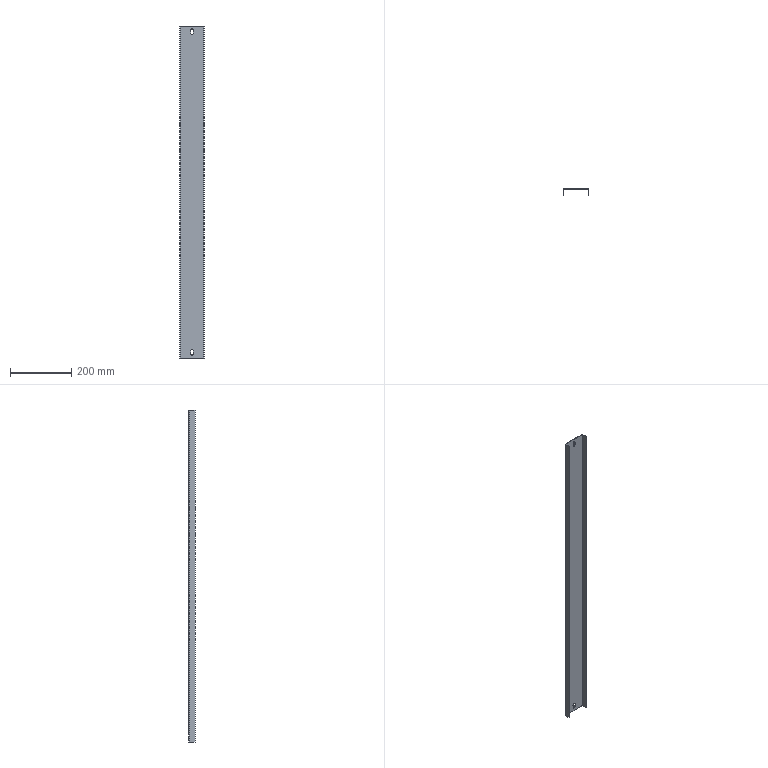Component | SolidWorks | MountingPlate-1 | 1 solid | 32 faces | box 81.5 x 20 x 1085 mm | volume 191237 mm3 | plane 22 | cylinder 10 | commonest cylinder face diameters 9 x6 3.2 x2 0.2 x2
STEP:
#1=COLOUR_RGB('',0.7922,0.8196,0.9333);
#2=FILL_AREA_STYLE_COLOUR('',#1);
#3=FILL_AREA_STYLE('',(#2));
#4=SURFACE_STYLE_FILL_AREA(#3);
#5=SURFACE_SIDE_STYLE('',(#4));
#6=SURFACE_STYLE_USAGE(.BOTH.,#5);
#7=PRESENTATION_STYLE_ASSIGNMENT((#6));
#8=CARTESIAN_POINT('',(11.302,-36.434,95.784));
#9=VERTEX_POINT('',#8);
#10=CARTESIAN_POINT('',(11.125,-36.434,95.607));
#11=VERTEX_POINT('',#10);
#12=CARTESIAN_POINT('',(11.302,-36.434,95.607));
#13=DIRECTION('',(0.,-1.,-0.));
#14=DIRECTION('',(0.,0.,1.));
#15=AXIS2_PLACEMENT_3D('',#12,#13,#14);
#16=CIRCLE('',#15,0.1772);
#17=EDGE_CURVE('',#9,#11,#16,.T.);
#18=ORIENTED_EDGE('',*,*,#17,.F.);
#19=CARTESIAN_POINT('',(11.302,-36.493,95.784));
#20=VERTEX_POINT('',#19);
#21=CARTESIAN_POINT('',(11.302,-36.434,95.784));
#22=DIRECTION('',(0.,-1.,-0.));
#23=VECTOR('',#22,39.37);
#24=LINE('',#21,#23);
#25=EDGE_CURVE('',#9,#20,#24,.T.);
#26=ORIENTED_EDGE('',*,*,#25,.T.);
#27=CARTESIAN_POINT('',(11.125,-36.493,95.607));
#28=VERTEX_POINT('',#27);
#29=CARTESIAN_POINT('',(11.302,-36.493,95.607));
#30=DIRECTION('',(0.,-1.,-0.));
#31=DIRECTION('',(0.,0.,1.));
#32=AXIS2_PLACEMENT_3D('',#29,#30,#31);
#33=CIRCLE('',#32,0.1772);
#34=EDGE_CURVE('',#20,#28,#33,.T.);
#35=ORIENTED_EDGE('',*,*,#34,.T.);
#36=CARTESIAN_POINT('',(11.125,-36.434,95.607));
#37=DIRECTION('',(0.,-1.,-0.));
#38=VECTOR('',#37,39.37);
#39=LINE('',#36,#38);
#40=EDGE_CURVE('',#11,#28,#39,.T.);
#41=ORIENTED_EDGE('',*,*,#40,.F.);
#42=EDGE_LOOP('',(#18,#26,#35,#41));
#43=FACE_OUTER_BOUND('',#42,.T.);
#44=CARTESIAN_POINT('',(11.302,-36.434,95.607));
#45=DIRECTION('',(0.,-1.,-0.));
#46=DIRECTION('',(0.,0.,1.));
#47=AXIS2_PLACEMENT_3D('',#44,#45,#46);
#48=CYLINDRICAL_SURFACE('',#47,0.1772);
#49=ADVANCED_FACE('',(#43),#48,.F.);
#50=CARTESIAN_POINT('',(11.302,-36.434,54.532));
#51=VERTEX_POINT('',#50);
#52=CARTESIAN_POINT('',(11.125,-36.434,54.355));
#53=VERTEX_POINT('',#52);
#54=CARTESIAN_POINT('',(11.302,-36.434,54.355));
#55=DIRECTION('',(0.,-1.,-0.));
#56=DIRECTION('',(0.,0.,1.));
#57=AXIS2_PLACEMENT_3D('',#54,#55,#56);
#58=CIRCLE('',#57,0.1772);
#59=EDGE_CURVE('',#51,#53,#58,.T.);
#60=ORIENTED_EDGE('',*,*,#59,.F.);
#61=CARTESIAN_POINT('',(11.302,-36.493,54.532));
#62=VERTEX_POINT('',#61);
#63=CARTESIAN_POINT('',(11.302,-36.434,54.532));
#64=DIRECTION('',(0.,-1.,-0.));
#65=VECTOR('',#64,39.37);
#66=LINE('',#63,#65);
#67=EDGE_CURVE('',#51,#62,#66,.T.);
#68=ORIENTED_EDGE('',*,*,#67,.T.);
#69=CARTESIAN_POINT('',(11.125,-36.493,54.355));
#70=VERTEX_POINT('',#69);
#71=CARTESIAN_POINT('',(11.302,-36.493,54.355));
#72=DIRECTION('',(0.,-1.,-0.));
#73=DIRECTION('',(0.,0.,1.));
#74=AXIS2_PLACEMENT_3D('',#71,#72,#73);
#75=CIRCLE('',#74,0.1772);
#76=EDGE_CURVE('',#62,#70,#75,.T.);
#77=ORIENTED_EDGE('',*,*,#76,.T.);
#78=CARTESIAN_POINT('',(11.125,-36.434,54.355));
#79=DIRECTION('',(0.,-1.,-0.));
#80=VECTOR('',#79,39.37);
#81=LINE('',#78,#80);
#82=EDGE_CURVE('',#53,#70,#81,.T.);
#83=ORIENTED_EDGE('',*,*,#82,.F.);
#84=EDGE_LOOP('',(#60,#68,#77,#83));
#85=FACE_OUTER_BOUND('',#84,.T.);
#86=CARTESIAN_POINT('',(11.302,-36.434,54.355));
#87=DIRECTION('',(0.,-1.,-0.));
#88=DIRECTION('',(0.,0.,1.));
#89=AXIS2_PLACEMENT_3D('',#86,#87,#88);
#90=CYLINDRICAL_SURFACE('',#89,0.1772);
#91=ADVANCED_FACE('',(#85),#90,.F.);
#92=CARTESIAN_POINT('',(11.48,-36.493,54.));
#93=VERTEX_POINT('',#92);
#94=CARTESIAN_POINT('',(11.48,-36.493,54.355));
#95=VERTEX_POINT('',#94);
#96=CARTESIAN_POINT('',(11.48,-36.493,54.355));
#97=DIRECTION('',(0.,-0.,1.));
#98=VECTOR('',#97,39.37);
#99=LINE('',#96,#98);
#100=EDGE_CURVE('',#93,#95,#99,.T.);
#101=ORIENTED_EDGE('',*,*,#100,.F.);
#102=CARTESIAN_POINT('',(11.125,-36.493,54.));
#103=VERTEX_POINT('',#102);
#104=CARTESIAN_POINT('',(11.302,-36.493,54.));
#105=DIRECTION('',(0.,-1.,-0.));
#106=DIRECTION('',(0.,0.,1.));
#107=AXIS2_PLACEMENT_3D('',#104,#105,#106);
#108=CIRCLE('',#107,0.1772);
#109=EDGE_CURVE('',#103,#93,#108,.T.);
#110=ORIENTED_EDGE('',*,*,#109,.F.);
#111=CARTESIAN_POINT('',(11.125,-36.493,54.355));
#112=DIRECTION('',(-0.,0.,-1.));
#113=VECTOR('',#112,39.37);
#114=LINE('',#111,#113);
#115=EDGE_CURVE('',#70,#103,#114,.T.);
#116=ORIENTED_EDGE('',*,*,#115,.F.);
#117=ORIENTED_EDGE('',*,*,#76,.F.);
#118=CARTESIAN_POINT('',(11.302,-36.493,54.355));
#119=DIRECTION('',(0.,-1.,-0.));
#120=DIRECTION('',(0.,0.,1.));
#121=AXIS2_PLACEMENT_3D('',#118,#119,#120);
#122=CIRCLE('',#121,0.1772);
#123=EDGE_CURVE('',#95,#62,#122,.T.);
#124=ORIENTED_EDGE('',*,*,#123,.F.);
#125=EDGE_LOOP('',(#101,#110,#116,#117,#124));
#126=FACE_BOUND('',#125,.T.);
#127=CARTESIAN_POINT('',(11.48,-36.493,95.252));
#128=VERTEX_POINT('',#127);
#129=CARTESIAN_POINT('',(11.48,-36.493,95.607));
#130=VERTEX_POINT('',#129);
#131=CARTESIAN_POINT('',(11.48,-36.493,95.607));
#132=DIRECTION('',(-0.,-0.,1.));
#133=VECTOR('',#132,39.37);
#134=LINE('',#131,#133);
#135=EDGE_CURVE('',#128,#130,#134,.T.);
#136=ORIENTED_EDGE('',*,*,#135,.F.);
#137=CARTESIAN_POINT('',(11.125,-36.493,95.252));
#138=VERTEX_POINT('',#137);
#139=CARTESIAN_POINT('',(11.302,-36.493,95.252));
#140=DIRECTION('',(0.,-1.,-0.));
#141=DIRECTION('',(0.,0.,1.));
#142=AXIS2_PLACEMENT_3D('',#139,#140,#141);
#143=CIRCLE('',#142,0.1772);
#144=EDGE_CURVE('',#138,#128,#143,.T.);
#145=ORIENTED_EDGE('',*,*,#144,.F.);
#146=CARTESIAN_POINT('',(11.125,-36.493,95.607));
#147=DIRECTION('',(-0.,0.,-1.));
#148=VECTOR('',#147,39.37);
#149=LINE('',#146,#148);
#150=EDGE_CURVE('',#28,#138,#149,.T.);
#151=ORIENTED_EDGE('',*,*,#150,.F.);
#152=ORIENTED_EDGE('',*,*,#34,.F.);
#153=CARTESIAN_POINT('',(11.302,-36.493,95.607));
#154=DIRECTION('',(0.,-1.,-0.));
#155=DIRECTION('',(0.,0.,1.));
#156=AXIS2_PLACEMENT_3D('',#153,#154,#155);
#157=CIRCLE('',#156,0.1772);
#158=EDGE_CURVE('',#130,#20,#157,.T.);
#159=ORIENTED_EDGE('',*,*,#158,.F.);
#160=EDGE_LOOP('',(#136,#145,#151,#152,#159));
#161=FACE_BOUND('',#160,.T.);
#162=CARTESIAN_POINT('',(9.761,-36.493,53.445));
#163=VERTEX_POINT('',#162);
#164=CARTESIAN_POINT('',(12.844,-36.493,53.445));
#165=VERTEX_POINT('',#164);
#166=CARTESIAN_POINT('',(13.604,-36.493,53.445));
#167=DIRECTION('',(1.,0.,-0.));
#168=VECTOR('',#167,39.37);
#169=LINE('',#166,#168);
#170=EDGE_CURVE('',#163,#165,#169,.T.);
#171=ORIENTED_EDGE('',*,*,#170,.T.);
#172=CARTESIAN_POINT('',(12.844,-36.493,96.162));
#173=VERTEX_POINT('',#172);
#174=CARTESIAN_POINT('',(12.844,-36.493,-1322.049));
#175=DIRECTION('',(0.,-0.,1.));
#176=VECTOR('',#175,39.37);
#177=LINE('',#174,#176);
#178=EDGE_CURVE('',#165,#173,#177,.T.);
#179=ORIENTED_EDGE('',*,*,#178,.T.);
#180=CARTESIAN_POINT('',(9.761,-36.493,96.162));
#181=VERTEX_POINT('',#180);
#182=CARTESIAN_POINT('',(9.001,-36.493,96.162));
#183=DIRECTION('',(-1.,-0.,0.));
#184=VECTOR('',#183,39.37);
#185=LINE('',#182,#184);
#186=EDGE_CURVE('',#173,#181,#185,.T.);
#187=ORIENTED_EDGE('',*,*,#186,.T.);
#188=CARTESIAN_POINT('',(9.761,-36.493,-1322.049));
#189=DIRECTION('',(0.,-0.,1.));
#190=VECTOR('',#189,39.37);
#191=LINE('',#188,#190);
#192=EDGE_CURVE('',#163,#181,#191,.T.);
#193=ORIENTED_EDGE('',*,*,#192,.F.);
#194=EDGE_LOOP('',(#171,#179,#187,#193));
#195=FACE_OUTER_BOUND('',#194,.T.);
#196=CARTESIAN_POINT('',(320.089,-36.493,-1322.049));
#197=DIRECTION('',(-0.,1.,0.));
#198=DIRECTION('',(-0.,0.,-1.));
#199=AXIS2_PLACEMENT_3D('',#196,#197,#198);
#200=PLANE('',#199);
#201=ADVANCED_FACE('',(#126,#161,#195),#200,.F.);
#202=CARTESIAN_POINT('',(12.844,-36.434,53.445));
#203=VERTEX_POINT('',#202);
#204=CARTESIAN_POINT('',(12.844,-36.434,53.445));
#205=DIRECTION('',(-0.,1.,0.));
#206=VECTOR('',#205,39.37);
#207=LINE('',#204,#206);
#208=EDGE_CURVE('',#165,#203,#207,.T.);
#209=ORIENTED_EDGE('',*,*,#208,.F.);
#210=ORIENTED_EDGE('',*,*,#170,.F.);
#211=CARTESIAN_POINT('',(9.761,-36.434,53.445));
#212=VERTEX_POINT('',#211);
#213=CARTESIAN_POINT('',(9.761,-36.434,53.445));
#214=DIRECTION('',(-0.,1.,0.));
#215=VECTOR('',#214,39.37);
#216=LINE('',#213,#215);
#217=EDGE_CURVE('',#163,#212,#216,.T.);
#218=ORIENTED_EDGE('',*,*,#217,.T.);
#219=CARTESIAN_POINT('',(13.604,-36.434,53.445));
#220=DIRECTION('',(1.,0.,-0.));
#221=VECTOR('',#220,39.37);
#222=LINE('',#219,#221);
#223=EDGE_CURVE('',#212,#203,#222,.T.);
#224=ORIENTED_EDGE('',*,*,#223,.T.);
#225=EDGE_LOOP('',(#209,#210,#218,#224));
#226=FACE_OUTER_BOUND('',#225,.T.);
#227=CARTESIAN_POINT('',(13.604,-36.434,53.445));
#228=DIRECTION('',(-0.,0.,-1.));
#229=DIRECTION('',(0.,-1.,-0.));
#230=AXIS2_PLACEMENT_3D('',#227,#228,#229);
#231=PLANE('',#230);
#232=ADVANCED_FACE('',(#226),#231,.T.);
#233=CARTESIAN_POINT('',(12.844,-36.434,96.162));
#234=VERTEX_POINT('',#233);
#235=CARTESIAN_POINT('',(12.844,-36.434,96.162));
#236=DIRECTION('',(0.,-1.,-0.));
#237=VECTOR('',#236,39.37);
#238=LINE('',#235,#237);
#239=EDGE_CURVE('',#234,#173,#238,.T.);
#240=ORIENTED_EDGE('',*,*,#239,.F.);
#241=CARTESIAN_POINT('',(9.761,-36.434,96.162));
#242=VERTEX_POINT('',#241);
#243=CARTESIAN_POINT('',(9.001,-36.434,96.162));
#244=DIRECTION('',(-1.,-0.,0.));
#245=VECTOR('',#244,39.37);
#246=LINE('',#243,#245);
#247=EDGE_CURVE('',#234,#242,#246,.T.);
#248=ORIENTED_EDGE('',*,*,#247,.T.);
#249=CARTESIAN_POINT('',(9.761,-36.434,96.162));
#250=DIRECTION('',(0.,-1.,-0.));
#251=VECTOR('',#250,39.37);
#252=LINE('',#249,#251);
#253=EDGE_CURVE('',#242,#181,#252,.T.);
#254=ORIENTED_EDGE('',*,*,#253,.T.);
#255=ORIENTED_EDGE('',*,*,#186,.F.);
#256=EDGE_LOOP('',(#240,#248,#254,#255));
#257=FACE_OUTER_BOUND('',#256,.T.);
#258=CARTESIAN_POINT('',(9.001,-36.434,96.162));
#259=DIRECTION('',(0.,-0.,1.));
#260=DIRECTION('',(-0.,1.,0.));
#261=AXIS2_PLACEMENT_3D('',#258,#259,#260);
#262=PLANE('',#261);
#263=ADVANCED_FACE('',(#257),#262,.T.);
#264=CARTESIAN_POINT('',(12.844,-36.434,-1322.049));
#265=DIRECTION('',(0.,-0.,1.));
#266=VECTOR('',#265,39.37);
#267=LINE('',#264,#266);
#268=EDGE_CURVE('',#203,#234,#267,.T.);
#269=ORIENTED_EDGE('',*,*,#268,.F.);
#270=ORIENTED_EDGE('',*,*,#223,.F.);
#271=CARTESIAN_POINT('',(9.761,-36.434,-1322.049));
#272=DIRECTION('',(0.,-0.,1.));
#273=VECTOR('',#272,39.37);
#274=LINE('',#271,#273);
#275=EDGE_CURVE('',#212,#242,#274,.T.);
#276=ORIENTED_EDGE('',*,*,#275,.T.);
#277=ORIENTED_EDGE('',*,*,#247,.F.);
#278=EDGE_LOOP('',(#269,#270,#276,#277));
#279=FACE_OUTER_BOUND('',#278,.T.);
#280=CARTESIAN_POINT('',(11.125,-36.434,95.252));
#281=VERTEX_POINT('',#280);
#282=CARTESIAN_POINT('',(11.48,-36.434,95.252));
#283=VERTEX_POINT('',#282);
#284=CARTESIAN_POINT('',(11.302,-36.434,95.252));
#285=DIRECTION('',(0.,-1.,-0.));
#286=DIRECTION('',(0.,0.,1.));
#287=AXIS2_PLACEMENT_3D('',#284,#285,#286);
#288=CIRCLE('',#287,0.1772);
#289=EDGE_CURVE('',#281,#283,#288,.T.);
#290=ORIENTED_EDGE('',*,*,#289,.T.);
#291=CARTESIAN_POINT('',(11.48,-36.434,95.607));
#292=VERTEX_POINT('',#291);
#293=CARTESIAN_POINT('',(11.48,-36.434,95.607));
#294=DIRECTION('',(-0.,-0.,1.));
#295=VECTOR('',#294,39.37);
#296=LINE('',#293,#295);
#297=EDGE_CURVE('',#283,#292,#296,.T.);
#298=ORIENTED_EDGE('',*,*,#297,.T.);
#299=CARTESIAN_POINT('',(11.302,-36.434,95.607));
#300=DIRECTION('',(0.,-1.,-0.));
#301=DIRECTION('',(0.,0.,1.));
#302=AXIS2_PLACEMENT_3D('',#299,#300,#301);
#303=CIRCLE('',#302,0.1772);
#304=EDGE_CURVE('',#292,#9,#303,.T.);
#305=ORIENTED_EDGE('',*,*,#304,.T.);
#306=ORIENTED_EDGE('',*,*,#17,.T.);
#307=CARTESIAN_POINT('',(11.125,-36.434,95.607));
#308=DIRECTION('',(-0.,0.,-1.));
#309=VECTOR('',#308,39.37);
#310=LINE('',#307,#309);
#311=EDGE_CURVE('',#11,#281,#310,.T.);
#312=ORIENTED_EDGE('',*,*,#311,.T.);
#313=EDGE_LOOP('',(#290,#298,#305,#306,#312));
#314=FACE_BOUND('',#313,.T.);
#315=CARTESIAN_POINT('',(11.125,-36.434,54.));
#316=VERTEX_POINT('',#315);
#317=CARTESIAN_POINT('',(11.48,-36.434,54.));
#318=VERTEX_POINT('',#317);
#319=CARTESIAN_POINT('',(11.302,-36.434,54.));
#320=DIRECTION('',(0.,-1.,-0.));
#321=DIRECTION('',(0.,0.,1.));
#322=AXIS2_PLACEMENT_3D('',#319,#320,#321);
#323=CIRCLE('',#322,0.1772);
#324=EDGE_CURVE('',#316,#318,#323,.T.);
#325=ORIENTED_EDGE('',*,*,#324,.T.);
#326=CARTESIAN_POINT('',(11.48,-36.434,54.355));
#327=VERTEX_POINT('',#326);
#328=CARTESIAN_POINT('',(11.48,-36.434,54.355));
#329=DIRECTION('',(0.,-0.,1.));
#330=VECTOR('',#329,39.37);
#331=LINE('',#328,#330);
#332=EDGE_CURVE('',#318,#327,#331,.T.);
#333=ORIENTED_EDGE('',*,*,#332,.T.);
#334=CARTESIAN_POINT('',(11.302,-36.434,54.355));
#335=DIRECTION('',(0.,-1.,-0.));
#336=DIRECTION('',(0.,0.,1.));
#337=AXIS2_PLACEMENT_3D('',#334,#335,#336);
#338=CIRCLE('',#337,0.1772);
#339=EDGE_CURVE('',#327,#51,#338,.T.);
#340=ORIENTED_EDGE('',*,*,#339,.T.);
#341=ORIENTED_EDGE('',*,*,#59,.T.);
#342=CARTESIAN_POINT('',(11.125,-36.434,54.355));
#343=DIRECTION('',(-0.,0.,-1.));
#344=VECTOR('',#343,39.37);
#345=LINE('',#342,#344);
#346=EDGE_CURVE('',#53,#316,#345,.T.);
#347=ORIENTED_EDGE('',*,*,#346,.T.);
#348=EDGE_LOOP('',(#325,#333,#340,#341,#347));
#349=FACE_BOUND('',#348,.T.);
#350=CARTESIAN_POINT('',(320.089,-36.434,-1322.049));
#351=DIRECTION('',(-0.,1.,0.));
#352=DIRECTION('',(-0.,0.,-1.));
#353=AXIS2_PLACEMENT_3D('',#350,#351,#352);
#354=PLANE('',#353);
#355=ADVANCED_FACE('',(#279,#314,#349),#354,.T.);
#356=ORIENTED_EDGE('',*,*,#109,.T.);
#357=CARTESIAN_POINT('',(11.48,-36.434,54.));
#358=DIRECTION('',(0.,-1.,-0.));
#359=VECTOR('',#358,39.37);
#360=LINE('',#357,#359);
#361=EDGE_CURVE('',#318,#93,#360,.T.);
#362=ORIENTED_EDGE('',*,*,#361,.F.);
#363=ORIENTED_EDGE('',*,*,#324,.F.);
#364=CARTESIAN_POINT('',(11.125,-36.434,54.));
#365=DIRECTION('',(0.,-1.,-0.));
#366=VECTOR('',#365,39.37);
#367=LINE('',#364,#366);
#368=EDGE_CURVE('',#316,#103,#367,.T.);
#369=ORIENTED_EDGE('',*,*,#368,.T.);
#370=EDGE_LOOP('',(#356,#362,#363,#369));
#371=FACE_OUTER_BOUND('',#370,.T.);
#372=CARTESIAN_POINT('',(11.302,-36.434,54.));
#373=DIRECTION('',(0.,-1.,-0.));
#374=DIRECTION('',(0.,0.,1.));
#375=AXIS2_PLACEMENT_3D('',#372,#373,#374);
#376=CYLINDRICAL_SURFACE('',#375,0.1772);
#377=ADVANCED_FACE('',(#371),#376,.F.);
#378=ORIENTED_EDGE('',*,*,#115,.T.);
#379=ORIENTED_EDGE('',*,*,#368,.F.);
#380=ORIENTED_EDGE('',*,*,#346,.F.);
#381=ORIENTED_EDGE('',*,*,#82,.T.);
#382=EDGE_LOOP('',(#378,#379,#380,#381));
#383=FACE_OUTER_BOUND('',#382,.T.);
#384=CARTESIAN_POINT('',(11.125,-36.434,54.355));
#385=DIRECTION('',(-1.,-0.,0.));
#386=DIRECTION('',(0.,-1.,-0.));
#387=AXIS2_PLACEMENT_3D('',#384,#385,#386);
#388=PLANE('',#387);
#389=ADVANCED_FACE('',(#383),#388,.F.);
#390=ORIENTED_EDGE('',*,*,#67,.F.);
#391=ORIENTED_EDGE('',*,*,#339,.F.);
#392=CARTESIAN_POINT('',(11.48,-36.434,54.355));
#393=DIRECTION('',(0.,-1.,-0.));
#394=VECTOR('',#393,39.37);
#395=LINE('',#392,#394);
#396=EDGE_CURVE('',#327,#95,#395,.T.);
#397=ORIENTED_EDGE('',*,*,#396,.T.);
#398=ORIENTED_EDGE('',*,*,#123,.T.);
#399=EDGE_LOOP('',(#390,#391,#397,#398));
#400=FACE_OUTER_BOUND('',#399,.T.);
#401=CARTESIAN_POINT('',(11.302,-36.434,54.355));
#402=DIRECTION('',(0.,-1.,-0.));
#403=DIRECTION('',(0.,0.,1.));
#404=AXIS2_PLACEMENT_3D('',#401,#402,#403);
#405=CYLINDRICAL_SURFACE('',#404,0.1772);
#406=ADVANCED_FACE('',(#400),#405,.F.);
#407=ORIENTED_EDGE('',*,*,#100,.T.);
#408=ORIENTED_EDGE('',*,*,#396,.F.);
#409=ORIENTED_EDGE('',*,*,#332,.F.);
#410=ORIENTED_EDGE('',*,*,#361,.T.);
#411=EDGE_LOOP('',(#407,#408,#409,#410));
#412=FACE_OUTER_BOUND('',#411,.T.);
#413=CARTESIAN_POINT('',(11.48,-36.434,54.355));
#414=DIRECTION('',(1.,0.,-0.));
#415=DIRECTION('',(-0.,1.,0.));
#416=AXIS2_PLACEMENT_3D('',#413,#414,#415);
#417=PLANE('',#416);
#418=ADVANCED_FACE('',(#412),#417,.F.);
#419=ORIENTED_EDGE('',*,*,#144,.T.);
#420=CARTESIAN_POINT('',(11.48,-36.434,95.252));
#421=DIRECTION('',(0.,-1.,-0.));
#422=VECTOR('',#421,39.37);
#423=LINE('',#420,#422);
#424=EDGE_CURVE('',#283,#128,#423,.T.);
#425=ORIENTED_EDGE('',*,*,#424,.F.);
#426=ORIENTED_EDGE('',*,*,#289,.F.);
#427=CARTESIAN_POINT('',(11.125,-36.434,95.252));
#428=DIRECTION('',(0.,-1.,-0.));
#429=VECTOR('',#428,39.37);
#430=LINE('',#427,#429);
#431=EDGE_CURVE('',#281,#138,#430,.T.);
#432=ORIENTED_EDGE('',*,*,#431,.T.);
#433=EDGE_LOOP('',(#419,#425,#426,#432));
#434=FACE_OUTER_BOUND('',#433,.T.);
#435=CARTESIAN_POINT('',(11.302,-36.434,95.252));
#436=DIRECTION('',(0.,-1.,-0.));
#437=DIRECTION('',(0.,0.,1.));
#438=AXIS2_PLACEMENT_3D('',#435,#436,#437);
#439=CYLINDRICAL_SURFACE('',#438,0.1772);
#440=ADVANCED_FACE('',(#434),#439,.F.);
#441=ORIENTED_EDGE('',*,*,#150,.T.);
#442=ORIENTED_EDGE('',*,*,#431,.F.);
#443=ORIENTED_EDGE('',*,*,#311,.F.);
#444=ORIENTED_EDGE('',*,*,#40,.T.);
#445=EDGE_LOOP('',(#441,#442,#443,#444));
#446=FACE_OUTER_BOUND('',#445,.T.);
#447=CARTESIAN_POINT('',(11.125,-36.434,95.607));
#448=DIRECTION('',(-1.,-0.,0.));
#449=DIRECTION('',(0.,-1.,-0.));
#450=AXIS2_PLACEMENT_3D('',#447,#448,#449);
#451=PLANE('',#450);
#452=ADVANCED_FACE('',(#446),#451,.F.);
#453=ORIENTED_EDGE('',*,*,#25,.F.);
#454=ORIENTED_EDGE('',*,*,#304,.F.);
#455=CARTESIAN_POINT('',(11.48,-36.434,95.607));
#456=DIRECTION('',(0.,-1.,-0.));
#457=VECTOR('',#456,39.37);
#458=LINE('',#455,#457);
#459=EDGE_CURVE('',#292,#130,#458,.T.);
#460=ORIENTED_EDGE('',*,*,#459,.T.);
#461=ORIENTED_EDGE('',*,*,#158,.T.);
#462=EDGE_LOOP('',(#453,#454,#460,#461));
#463=FACE_OUTER_BOUND('',#462,.T.);
#464=CARTESIAN_POINT('',(11.302,-36.434,95.607));
#465=DIRECTION('',(0.,-1.,-0.));
#466=DIRECTION('',(0.,0.,1.));
#467=AXIS2_PLACEMENT_3D('',#464,#465,#466);
#468=CYLINDRICAL_SURFACE('',#467,0.1772);
#469=ADVANCED_FACE('',(#463),#468,.F.);
#470=ORIENTED_EDGE('',*,*,#135,.T.);
#471=ORIENTED_EDGE('',*,*,#459,.F.);
#472=ORIENTED_EDGE('',*,*,#297,.F.);
#473=ORIENTED_EDGE('',*,*,#424,.T.);
#474=EDGE_LOOP('',(#470,#471,#472,#473));
#475=FACE_OUTER_BOUND('',#474,.T.);
#476=CARTESIAN_POINT('',(11.48,-36.434,95.607));
#477=DIRECTION('',(1.,0.,0.));
#478=DIRECTION('',(-0.,-0.,1.));
#479=AXIS2_PLACEMENT_3D('',#476,#477,#478);
#480=PLANE('',#479);
#481=ADVANCED_FACE('',(#475),#480,.F.);
#482=ORIENTED_EDGE('',*,*,#217,.F.);
#483=CARTESIAN_POINT('',(9.757,-36.497,53.445));
#484=VERTEX_POINT('',#483);
#485=CARTESIAN_POINT('',(9.761,-36.497,53.445));
#486=DIRECTION('',(0.,-0.,1.));
#487=DIRECTION('',(0.,1.,0.));
#488=AXIS2_PLACEMENT_3D('',#485,#486,#487);
#489=CIRCLE('',#488,0.003937);
#490=EDGE_CURVE('',#163,#484,#489,.T.);
#491=ORIENTED_EDGE('',*,*,#490,.T.);
#492=CARTESIAN_POINT('',(9.698,-36.497,53.445));
#493=VERTEX_POINT('',#492);
#494=CARTESIAN_POINT('',(9.698,-36.497,53.445));
#495=DIRECTION('',(-1.,-0.,0.));
#496=VECTOR('',#495,39.37);
#497=LINE('',#494,#496);
#498=EDGE_CURVE('',#484,#493,#497,.T.);
#499=ORIENTED_EDGE('',*,*,#498,.T.);
#500=CARTESIAN_POINT('',(9.761,-36.497,53.445));
#501=DIRECTION('',(0.,-0.,1.));
#502=DIRECTION('',(0.,-1.,0.));
#503=AXIS2_PLACEMENT_3D('',#500,#501,#502);
#504=CIRCLE('',#503,0.06299);
#505=EDGE_CURVE('',#212,#493,#504,.T.);
#506=ORIENTED_EDGE('',*,*,#505,.F.);
#507=EDGE_LOOP('',(#482,#491,#499,#506));
#508=FACE_OUTER_BOUND('',#507,.T.);
#509=CARTESIAN_POINT('',(9.761,-36.497,53.445));
#510=DIRECTION('',(-0.,0.,-1.));
#511=DIRECTION('',(0.,-1.,-0.));
#512=AXIS2_PLACEMENT_3D('',#509,#510,#511);
#513=PLANE('',#512);
#514=ADVANCED_FACE('',(#508),#513,.T.);
#515=CARTESIAN_POINT('',(9.757,-36.497,96.162));
#516=VERTEX_POINT('',#515);
#517=CARTESIAN_POINT('',(9.761,-36.497,96.162));
#518=DIRECTION('',(-0.,0.,-1.));
#519=DIRECTION('',(0.,1.,0.));
#520=AXIS2_PLACEMENT_3D('',#517,#518,#519);
#521=CIRCLE('',#520,0.003937);
#522=EDGE_CURVE('',#516,#181,#521,.T.);
#523=ORIENTED_EDGE('',*,*,#522,.T.);
#524=ORIENTED_EDGE('',*,*,#253,.F.);
#525=CARTESIAN_POINT('',(9.698,-36.497,96.162));
#526=VERTEX_POINT('',#525);
#527=CARTESIAN_POINT('',(9.761,-36.497,96.162));
#528=DIRECTION('',(-0.,0.,-1.));
#529=DIRECTION('',(0.,1.,0.));
#530=AXIS2_PLACEMENT_3D('',#527,#528,#529);
#531=CIRCLE('',#530,0.06299);
#532=EDGE_CURVE('',#526,#242,#531,.T.);
#533=ORIENTED_EDGE('',*,*,#532,.F.);
#534=CARTESIAN_POINT('',(9.698,-36.497,96.162));
#535=DIRECTION('',(1.,0.,-0.));
#536=VECTOR('',#535,39.37);
#537=LINE('',#534,#536);
#538=EDGE_CURVE('',#526,#516,#537,.T.);
#539=ORIENTED_EDGE('',*,*,#538,.T.);
#540=EDGE_LOOP('',(#523,#524,#533,#539));
#541=FACE_OUTER_BOUND('',#540,.T.);
#542=CARTESIAN_POINT('',(9.761,-36.497,96.162));
#543=DIRECTION('',(0.,-0.,1.));
#544=DIRECTION('',(-0.,1.,0.));
#545=AXIS2_PLACEMENT_3D('',#542,#543,#544);
#546=PLANE('',#545);
#547=ADVANCED_FACE('',(#541),#546,.T.);
#548=CARTESIAN_POINT('',(9.698,-36.497,-1322.049));
#549=DIRECTION('',(0.,-0.,1.));
#550=VECTOR('',#549,39.37);
#551=LINE('',#548,#550);
#552=EDGE_CURVE('',#493,#526,#551,.T.);
#553=ORIENTED_EDGE('',*,*,#552,.T.);
#554=ORIENTED_EDGE('',*,*,#532,.T.);
#555=ORIENTED_EDGE('',*,*,#275,.F.);
#556=ORIENTED_EDGE('',*,*,#505,.T.);
#557=EDGE_LOOP('',(#553,#554,#555,#556));
#558=FACE_OUTER_BOUND('',#557,.T.);
#559=CARTESIAN_POINT('',(9.761,-36.497,32.087));
#560=DIRECTION('',(0.,-0.,1.));
#561=DIRECTION('',(0.,1.,0.));
#562=AXIS2_PLACEMENT_3D('',#559,#560,#561);
#563=CYLINDRICAL_SURFACE('',#562,0.06299);
#564=ADVANCED_FACE('',(#558),#563,.T.);
#565=CARTESIAN_POINT('',(9.757,-36.497,-1322.049));
#566=DIRECTION('',(0.,-0.,1.));
#567=VECTOR('',#566,39.37);
#568=LINE('',#565,#567);
#569=EDGE_CURVE('',#484,#516,#568,.T.);
#570=ORIENTED_EDGE('',*,*,#569,.F.);
#571=ORIENTED_EDGE('',*,*,#490,.F.);
#572=ORIENTED_EDGE('',*,*,#192,.T.);
#573=ORIENTED_EDGE('',*,*,#522,.F.);
#574=EDGE_LOOP('',(#570,#571,#572,#573));
#575=FACE_OUTER_BOUND('',#574,.T.);
#576=CARTESIAN_POINT('',(9.761,-36.497,32.087));
#577=DIRECTION('',(0.,-0.,1.));
#578=DIRECTION('',(0.,1.,0.));
#579=AXIS2_PLACEMENT_3D('',#576,#577,#578);
#580=CYLINDRICAL_SURFACE('',#579,0.003937);
#581=ADVANCED_FACE('',(#575),#580,.F.);
#582=CARTESIAN_POINT('',(9.757,-37.222,96.162));
#583=VERTEX_POINT('',#582);
#584=CARTESIAN_POINT('',(9.757,-37.222,53.445));
#585=VERTEX_POINT('',#584);
#586=CARTESIAN_POINT('',(9.757,-37.222,53.445));
#587=DIRECTION('',(-0.,0.,-1.));
#588=VECTOR('',#587,39.37);
#589=LINE('',#586,#588);
#590=EDGE_CURVE('',#583,#585,#589,.T.);
#591=ORIENTED_EDGE('',*,*,#590,.F.);
#592=CARTESIAN_POINT('',(9.698,-37.222,96.162));
#593=VERTEX_POINT('',#592);
#594=CARTESIAN_POINT('',(9.698,-37.222,96.162));
#595=DIRECTION('',(1.,0.,-0.));
#596=VECTOR('',#595,39.37);
#597=LINE('',#594,#596);
#598=EDGE_CURVE('',#593,#583,#597,.T.);
#599=ORIENTED_EDGE('',*,*,#598,.F.);
#600=CARTESIAN_POINT('',(9.698,-37.222,53.445));
#601=VERTEX_POINT('',#600);
#602=CARTESIAN_POINT('',(9.698,-37.222,53.445));
#603=DIRECTION('',(-0.,0.,-1.));
#604=VECTOR('',#603,39.37);
#605=LINE('',#602,#604);
#606=EDGE_CURVE('',#593,#601,#605,.T.);
#607=ORIENTED_EDGE('',*,*,#606,.T.);
#608=CARTESIAN_POINT('',(9.698,-37.222,53.445));
#609=DIRECTION('',(1.,0.,-0.));
#610=VECTOR('',#609,39.37);
#611=LINE('',#608,#610);
#612=EDGE_CURVE('',#601,#585,#611,.T.);
#613=ORIENTED_EDGE('',*,*,#612,.T.);
#614=EDGE_LOOP('',(#591,#599,#607,#613));
#615=FACE_OUTER_BOUND('',#614,.T.);
#616=CARTESIAN_POINT('',(9.698,-37.222,53.445));
#617=DIRECTION('',(0.,-1.,-0.));
#618=DIRECTION('',(1.,0.,-0.));
#619=AXIS2_PLACEMENT_3D('',#616,#617,#618);
#620=PLANE('',#619);
#621=ADVANCED_FACE('',(#615),#620,.T.);
#622=ORIENTED_EDGE('',*,*,#552,.F.);
#623=CARTESIAN_POINT('',(9.698,-32.619,53.445));
#624=DIRECTION('',(-0.,1.,0.));
#625=VECTOR('',#624,39.37);
#626=LINE('',#623,#625);
#627=EDGE_CURVE('',#601,#493,#626,.T.);
#628=ORIENTED_EDGE('',*,*,#627,.F.);
#629=ORIENTED_EDGE('',*,*,#606,.F.);
#630=CARTESIAN_POINT('',(9.698,-37.222,96.162));
#631=DIRECTION('',(0.,-1.,-0.));
#632=VECTOR('',#631,39.37);
#633=LINE('',#630,#632);
#634=EDGE_CURVE('',#526,#593,#633,.T.);
#635=ORIENTED_EDGE('',*,*,#634,.F.);
#636=EDGE_LOOP('',(#622,#628,#629,#635));
#637=FACE_OUTER_BOUND('',#636,.T.);
#638=CARTESIAN_POINT('',(9.698,273.867,-1322.049));
#639=DIRECTION('',(-1.,-0.,0.));
#640=DIRECTION('',(-0.,0.,-1.));
#641=AXIS2_PLACEMENT_3D('',#638,#639,#640);
#642=PLANE('',#641);
#643=ADVANCED_FACE('',(#637),#642,.T.);
#644=ORIENTED_EDGE('',*,*,#498,.F.);
#645=CARTESIAN_POINT('',(9.757,-32.619,53.445));
#646=DIRECTION('',(-0.,1.,0.));
#647=VECTOR('',#646,39.37);
#648=LINE('',#645,#647);
#649=EDGE_CURVE('',#585,#484,#648,.T.);
#650=ORIENTED_EDGE('',*,*,#649,.F.);
#651=ORIENTED_EDGE('',*,*,#612,.F.);
#652=ORIENTED_EDGE('',*,*,#627,.T.);
#653=EDGE_LOOP('',(#644,#650,#651,#652));
#654=FACE_OUTER_BOUND('',#653,.T.);
#655=CARTESIAN_POINT('',(9.698,-32.619,53.445));
#656=DIRECTION('',(-0.,0.,-1.));
#657=DIRECTION('',(1.,0.,-0.));
#658=AXIS2_PLACEMENT_3D('',#655,#656,#657);
#659=PLANE('',#658);
#660=ADVANCED_FACE('',(#654),#659,.T.);
#661=ORIENTED_EDGE('',*,*,#649,.T.);
#662=ORIENTED_EDGE('',*,*,#569,.T.);
#663=CARTESIAN_POINT('',(9.757,-37.222,96.162));
#664=DIRECTION('',(0.,-1.,-0.));
#665=VECTOR('',#664,39.37);
#666=LINE('',#663,#665);
#667=EDGE_CURVE('',#516,#583,#666,.T.);
#668=ORIENTED_EDGE('',*,*,#667,.T.);
#669=ORIENTED_EDGE('',*,*,#590,.T.);
#670=EDGE_LOOP('',(#661,#662,#668,#669));
#671=FACE_OUTER_BOUND('',#670,.T.);
#672=CARTESIAN_POINT('',(9.757,273.867,-1322.049));
#673=DIRECTION('',(-1.,-0.,0.));
#674=DIRECTION('',(-0.,0.,-1.));
#675=AXIS2_PLACEMENT_3D('',#672,#673,#674);
#676=PLANE('',#675);
#677=ADVANCED_FACE('',(#671),#676,.F.);
#678=ORIENTED_EDGE('',*,*,#538,.F.);
#679=ORIENTED_EDGE('',*,*,#634,.T.);
#680=ORIENTED_EDGE('',*,*,#598,.T.);
#681=ORIENTED_EDGE('',*,*,#667,.F.);
#682=EDGE_LOOP('',(#678,#679,#680,#681));
#683=FACE_OUTER_BOUND('',#682,.T.);
#684=CARTESIAN_POINT('',(9.698,-37.222,96.162));
#685=DIRECTION('',(0.,-0.,1.));
#686=DIRECTION('',(-1.,-0.,0.));
#687=AXIS2_PLACEMENT_3D('',#684,#685,#686);
#688=PLANE('',#687);
#689=ADVANCED_FACE('',(#683),#688,.T.);
#690=CARTESIAN_POINT('',(12.848,-36.497,53.445));
#691=VERTEX_POINT('',#690);
#692=CARTESIAN_POINT('',(12.907,-36.497,53.445));
#693=VERTEX_POINT('',#692);
#694=CARTESIAN_POINT('',(12.907,-36.497,53.445));
#695=DIRECTION('',(1.,0.,-0.));
#696=VECTOR('',#695,39.37);
#697=LINE('',#694,#696);
#698=EDGE_CURVE('',#691,#693,#697,.T.);
#699=ORIENTED_EDGE('',*,*,#698,.F.);
#700=CARTESIAN_POINT('',(12.844,-36.497,53.445));
#701=DIRECTION('',(0.,-0.,1.));
#702=DIRECTION('',(0.,-1.,0.));
#703=AXIS2_PLACEMENT_3D('',#700,#701,#702);
#704=CIRCLE('',#703,0.003937);
#705=EDGE_CURVE('',#691,#165,#704,.T.);
#706=ORIENTED_EDGE('',*,*,#705,.T.);
#707=ORIENTED_EDGE('',*,*,#208,.T.);
#708=CARTESIAN_POINT('',(12.844,-36.497,53.445));
#709=DIRECTION('',(0.,-0.,1.));
#710=DIRECTION('',(0.,-1.,0.));
#711=AXIS2_PLACEMENT_3D('',#708,#709,#710);
#712=CIRCLE('',#711,0.06299);
#713=EDGE_CURVE('',#693,#203,#712,.T.);
#714=ORIENTED_EDGE('',*,*,#713,.F.);
#715=EDGE_LOOP('',(#699,#706,#707,#714));
#716=FACE_OUTER_BOUND('',#715,.T.);
#717=CARTESIAN_POINT('',(12.844,-36.497,53.445));
#718=DIRECTION('',(-0.,0.,-1.));
#719=DIRECTION('',(0.,-1.,-0.));
#720=AXIS2_PLACEMENT_3D('',#717,#718,#719);
#721=PLANE('',#720);
#722=ADVANCED_FACE('',(#716),#721,.T.);
#723=CARTESIAN_POINT('',(12.848,-36.497,96.162));
#724=VERTEX_POINT('',#723);
#725=CARTESIAN_POINT('',(12.844,-36.497,96.162));
#726=DIRECTION('',(-0.,0.,-1.));
#727=DIRECTION('',(0.,-1.,0.));
#728=AXIS2_PLACEMENT_3D('',#725,#726,#727);
#729=CIRCLE('',#728,0.003937);
#730=EDGE_CURVE('',#173,#724,#729,.T.);
#731=ORIENTED_EDGE('',*,*,#730,.T.);
#732=CARTESIAN_POINT('',(12.907,-36.497,96.162));
#733=VERTEX_POINT('',#732);
#734=CARTESIAN_POINT('',(12.907,-36.497,96.162));
#735=DIRECTION('',(-1.,-0.,0.));
#736=VECTOR('',#735,39.37);
#737=LINE('',#734,#736);
#738=EDGE_CURVE('',#733,#724,#737,.T.);
#739=ORIENTED_EDGE('',*,*,#738,.F.);
#740=CARTESIAN_POINT('',(12.844,-36.497,96.162));
#741=DIRECTION('',(-0.,0.,-1.));
#742=DIRECTION('',(0.,1.,0.));
#743=AXIS2_PLACEMENT_3D('',#740,#741,#742);
#744=CIRCLE('',#743,0.06299);
#745=EDGE_CURVE('',#234,#733,#744,.T.);
#746=ORIENTED_EDGE('',*,*,#745,.F.);
#747=ORIENTED_EDGE('',*,*,#239,.T.);
#748=EDGE_LOOP('',(#731,#739,#746,#747));
#749=FACE_OUTER_BOUND('',#748,.T.);
#750=CARTESIAN_POINT('',(12.844,-36.497,96.162));
#751=DIRECTION('',(0.,-0.,1.));
#752=DIRECTION('',(-0.,1.,0.));
#753=AXIS2_PLACEMENT_3D('',#750,#751,#752);
#754=PLANE('',#753);
#755=ADVANCED_FACE('',(#749),#754,.T.);
#756=ORIENTED_EDGE('',*,*,#268,.T.);
#757=ORIENTED_EDGE('',*,*,#745,.T.);
#758=CARTESIAN_POINT('',(12.907,-36.497,-1322.049));
#759=DIRECTION('',(0.,-0.,1.));
#760=VECTOR('',#759,39.37);
#761=LINE('',#758,#760);
#762=EDGE_CURVE('',#693,#733,#761,.T.);
#763=ORIENTED_EDGE('',*,*,#762,.F.);
#764=ORIENTED_EDGE('',*,*,#713,.T.);
#765=EDGE_LOOP('',(#756,#757,#763,#764));
#766=FACE_OUTER_BOUND('',#765,.T.);
#767=CARTESIAN_POINT('',(12.844,-36.497,117.52));
#768=DIRECTION('',(-0.,0.,-1.));
#769=DIRECTION('',(0.,-1.,0.));
#770=AXIS2_PLACEMENT_3D('',#767,#768,#769);
#771=CYLINDRICAL_SURFACE('',#770,0.06299);
#772=ADVANCED_FACE('',(#766),#771,.T.);
#773=ORIENTED_EDGE('',*,*,#178,.F.);
#774=ORIENTED_EDGE('',*,*,#705,.F.);
#775=CARTESIAN_POINT('',(12.848,-36.497,-1322.049));
#776=DIRECTION('',(0.,-0.,1.));
#777=VECTOR('',#776,39.37);
#778=LINE('',#775,#777);
#779=EDGE_CURVE('',#691,#724,#778,.T.);
#780=ORIENTED_EDGE('',*,*,#779,.T.);
#781=ORIENTED_EDGE('',*,*,#730,.F.);
#782=EDGE_LOOP('',(#773,#774,#780,#781));
#783=FACE_OUTER_BOUND('',#782,.T.);
#784=CARTESIAN_POINT('',(12.844,-36.497,117.52));
#785=DIRECTION('',(-0.,0.,-1.));
#786=DIRECTION('',(0.,-1.,0.));
#787=AXIS2_PLACEMENT_3D('',#784,#785,#786);
#788=CYLINDRICAL_SURFACE('',#787,0.003937);
#789=ADVANCED_FACE('',(#783),#788,.F.);
#790=CARTESIAN_POINT('',(12.848,-37.222,53.445));
#791=VERTEX_POINT('',#790);
#792=CARTESIAN_POINT('',(12.848,-37.222,96.162));
#793=VERTEX_POINT('',#792);
#794=CARTESIAN_POINT('',(12.848,-37.222,96.162));
#795=DIRECTION('',(0.,-0.,1.));
#796=VECTOR('',#795,39.37);
#797=LINE('',#794,#796);
#798=EDGE_CURVE('',#791,#793,#797,.T.);
#799=ORIENTED_EDGE('',*,*,#798,.F.);
#800=CARTESIAN_POINT('',(12.907,-37.222,53.445));
#801=VERTEX_POINT('',#800);
#802=CARTESIAN_POINT('',(12.907,-37.222,53.445));
#803=DIRECTION('',(-1.,0.,0.));
#804=VECTOR('',#803,39.37);
#805=LINE('',#802,#804);
#806=EDGE_CURVE('',#801,#791,#805,.T.);
#807=ORIENTED_EDGE('',*,*,#806,.F.);
#808=CARTESIAN_POINT('',(12.907,-37.222,96.162));
#809=VERTEX_POINT('',#808);
#810=CARTESIAN_POINT('',(12.907,-37.222,96.162));
#811=DIRECTION('',(0.,-0.,1.));
#812=VECTOR('',#811,39.37);
#813=LINE('',#810,#812);
#814=EDGE_CURVE('',#801,#809,#813,.T.);
#815=ORIENTED_EDGE('',*,*,#814,.T.);
#816=CARTESIAN_POINT('',(12.907,-37.222,96.162));
#817=DIRECTION('',(-1.,0.,0.));
#818=VECTOR('',#817,39.37);
#819=LINE('',#816,#818);
#820=EDGE_CURVE('',#809,#793,#819,.T.);
#821=ORIENTED_EDGE('',*,*,#820,.T.);
#822=EDGE_LOOP('',(#799,#807,#815,#821));
#823=FACE_OUTER_BOUND('',#822,.T.);
#824=CARTESIAN_POINT('',(12.907,-37.222,96.162));
#825=DIRECTION('',(-0.,-1.,-0.));
#826=DIRECTION('',(1.,-0.,-0.));
#827=AXIS2_PLACEMENT_3D('',#824,#825,#826);
#828=PLANE('',#827);
#829=ADVANCED_FACE('',(#823),#828,.T.);
#830=CARTESIAN_POINT('',(12.907,-37.222,53.445));
#831=DIRECTION('',(-0.,-1.,-0.));
#832=VECTOR('',#831,39.37);
#833=LINE('',#830,#832);
#834=EDGE_CURVE('',#693,#801,#833,.T.);
#835=ORIENTED_EDGE('',*,*,#834,.F.);
#836=ORIENTED_EDGE('',*,*,#762,.T.);
#837=CARTESIAN_POINT('',(12.907,-32.619,96.162));
#838=DIRECTION('',(0.,1.,0.));
#839=VECTOR('',#838,39.37);
#840=LINE('',#837,#839);
#841=EDGE_CURVE('',#809,#733,#840,.T.);
#842=ORIENTED_EDGE('',*,*,#841,.F.);
#843=ORIENTED_EDGE('',*,*,#814,.F.);
#844=EDGE_LOOP('',(#835,#836,#842,#843));
#845=FACE_OUTER_BOUND('',#844,.T.);
#846=CARTESIAN_POINT('',(12.907,-343.707,-1322.049));
#847=DIRECTION('',(1.,-0.,-0.));
#848=DIRECTION('',(-0.,0.,-1.));
#849=AXIS2_PLACEMENT_3D('',#846,#847,#848);
#850=PLANE('',#849);
#851=ADVANCED_FACE('',(#845),#850,.T.);
#852=ORIENTED_EDGE('',*,*,#841,.T.);
#853=ORIENTED_EDGE('',*,*,#738,.T.);
#854=CARTESIAN_POINT('',(12.848,-32.619,96.162));
#855=DIRECTION('',(0.,1.,0.));
#856=VECTOR('',#855,39.37);
#857=LINE('',#854,#856);
#858=EDGE_CURVE('',#793,#724,#857,.T.);
#859=ORIENTED_EDGE('',*,*,#858,.F.);
#860=ORIENTED_EDGE('',*,*,#820,.F.);
#861=EDGE_LOOP('',(#852,#853,#859,#860));
#862=FACE_OUTER_BOUND('',#861,.T.);
#863=CARTESIAN_POINT('',(12.907,-32.619,96.162));
#864=DIRECTION('',(0.,-0.,1.));
#865=DIRECTION('',(1.,-0.,-0.));
#866=AXIS2_PLACEMENT_3D('',#863,#864,#865);
#867=PLANE('',#866);
#868=ADVANCED_FACE('',(#862),#867,.T.);
#869=ORIENTED_EDGE('',*,*,#779,.F.);
#870=CARTESIAN_POINT('',(12.848,-37.222,53.445));
#871=DIRECTION('',(-0.,-1.,-0.));
#872=VECTOR('',#871,39.37);
#873=LINE('',#870,#872);
#874=EDGE_CURVE('',#691,#791,#873,.T.);
#875=ORIENTED_EDGE('',*,*,#874,.T.);
#876=ORIENTED_EDGE('',*,*,#798,.T.);
#877=ORIENTED_EDGE('',*,*,#858,.T.);
#878=EDGE_LOOP('',(#869,#875,#876,#877));
#879=FACE_OUTER_BOUND('',#878,.T.);
#880=CARTESIAN_POINT('',(12.848,-343.707,-1322.049));
#881=DIRECTION('',(1.,-0.,-0.));
#882=DIRECTION('',(-0.,0.,-1.));
#883=AXIS2_PLACEMENT_3D('',#880,#881,#882);
#884=PLANE('',#883);
#885=ADVANCED_FACE('',(#879),#884,.F.);
#886=ORIENTED_EDGE('',*,*,#874,.F.);
#887=ORIENTED_EDGE('',*,*,#698,.T.);
#888=ORIENTED_EDGE('',*,*,#834,.T.);
#889=ORIENTED_EDGE('',*,*,#806,.T.);
#890=EDGE_LOOP('',(#886,#887,#888,#889));
#891=FACE_OUTER_BOUND('',#890,.T.);
#892=CARTESIAN_POINT('',(12.907,-37.222,53.445));
#893=DIRECTION('',(-0.,0.,-1.));
#894=DIRECTION('',(-1.,0.,0.));
#895=AXIS2_PLACEMENT_3D('',#892,#893,#894);
#896=PLANE('',#895);
#897=ADVANCED_FACE('',(#891),#896,.T.);
#898=CLOSED_SHELL('',(#49,#91,#201,#232,#263,#355,#377,#389,#406,#418,#440,#452,#469,#481,#514,#547,#564,#581,#621,#643,#660,#677,#689,#722,#755,#772,#789,#829,#851,#868,#885,#897));
#899=MANIFOLD_SOLID_BREP('',#898);
#900=STYLED_ITEM('',(#7),#899);
#901=PRESENTATION_LAYER_ASSIGNMENT('','',(#900));
#902=(LENGTH_UNIT()NAMED_UNIT(*)SI_UNIT($,.METRE.));
#903=LENGTH_MEASURE_WITH_UNIT(LENGTH_MEASURE(0.0254),#902);
#904=DIMENSIONAL_EXPONENTS(1.,0.,0.,0.,0.,0.,0.);
#905=(CONVERSION_BASED_UNIT('',#903)LENGTH_UNIT()NAMED_UNIT(#904));
#906=UNCERTAINTY_MEASURE_WITH_UNIT(LENGTH_MEASURE(0.00001),#905,'','');
#907=(NAMED_UNIT(*)PLANE_ANGLE_UNIT()SI_UNIT($,.RADIAN.));
#908=(NAMED_UNIT(*)SI_UNIT($,.STERADIAN.)SOLID_ANGLE_UNIT());
#909=(GEOMETRIC_REPRESENTATION_CONTEXT(3)GLOBAL_UNCERTAINTY_ASSIGNED_CONTEXT((#906))GLOBAL_UNIT_ASSIGNED_CONTEXT((#905,#907,#908))REPRESENTATION_CONTEXT('',''));
#910=MECHANICAL_DESIGN_GEOMETRIC_PRESENTATION_REPRESENTATION('',(#900),#909);
#911=CARTESIAN_POINT('',(0.,0.,0.));
#912=DIRECTION('',(0.,0.,1.));
#913=DIRECTION('',(1.,0.,0.));
#914=AXIS2_PLACEMENT_3D('',#911,#912,#913);
#915=(LENGTH_UNIT()NAMED_UNIT(*)SI_UNIT($,.METRE.));
#916=LENGTH_MEASURE_WITH_UNIT(LENGTH_MEASURE(0.0254),#915);
#917=DIMENSIONAL_EXPONENTS(1.,0.,0.,0.,0.,0.,0.);
#918=(CONVERSION_BASED_UNIT('',#916)LENGTH_UNIT()NAMED_UNIT(#917));
#919=UNCERTAINTY_MEASURE_WITH_UNIT(LENGTH_MEASURE(0.00001),#918,'','');
#920=(NAMED_UNIT(*)PLANE_ANGLE_UNIT()SI_UNIT($,.RADIAN.));
#921=(NAMED_UNIT(*)SI_UNIT($,.STERADIAN.)SOLID_ANGLE_UNIT());
#922=(GEOMETRIC_REPRESENTATION_CONTEXT(3)GLOBAL_UNCERTAINTY_ASSIGNED_CONTEXT((#919))GLOBAL_UNIT_ASSIGNED_CONTEXT((#918,#920,#921))REPRESENTATION_CONTEXT('',''));
#923=ADVANCED_BREP_SHAPE_REPRESENTATION('',(#899,#914),#922);